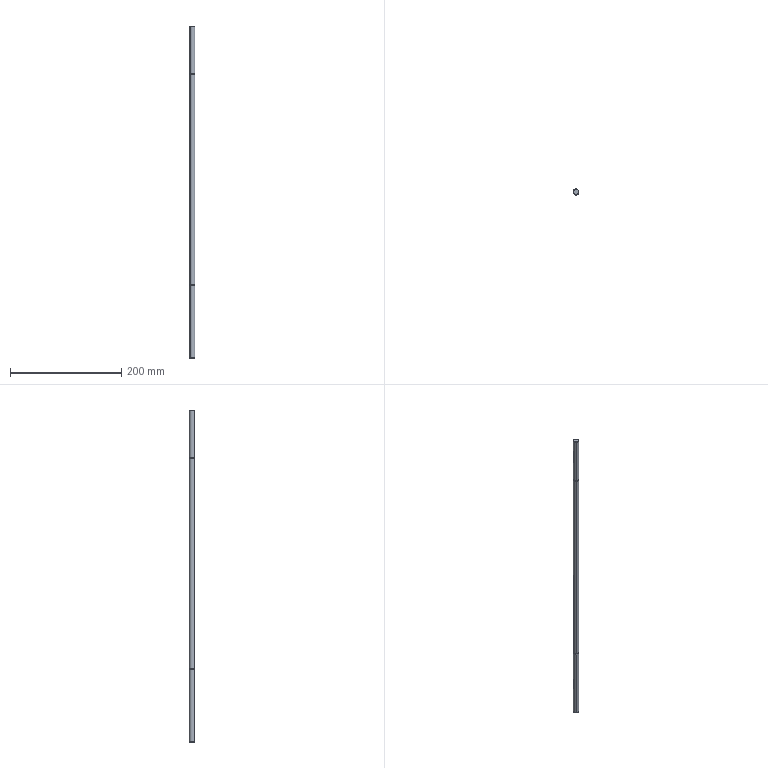Component | SolidWorks | LongGearAxis-1 | 1 solid | 20 faces | box 10 x 10 x 598 mm | volume 46949 mm3 | cylinder 10 | plane 6 | cone 4 | commonest cylinder face diameters 10 x6 9.7 x4
build123d program:
from build123d import *


with BuildPart() as part:
    # Sketch1 → Revolve1 (revolve)
    with BuildSketch(Plane.XY, mode=Mode.PRIVATE) as revolve1_sk:
        Polygon((-299, 4.5), (-299, 0), (299, 0), (299, 4.5), (298.5, 5), (168.6, 5), (168.6, 4.85), (167.5, 4.85), (167.5, 5), (-212.5, 5), (-212.5, 4.85), (-213.6, 4.85), (-213.6, 5), (-298.5, 5), align=None)
    revolve(revolve1_sk.sketch.rotate(Axis((-299, 0, 0), (1, 0, 0)), 270), axis=Axis((-299, 0, 0), (1, 0, 0)))


solid = part.part

# Placed as in the assembly
solid = solid.moved(Location((-180.767, 560.9, -22.5), (0, 90, 0)))
STEP:
#1=CARTESIAN_POINT('',(-7.025,22.234,-12.657));
#2=VERTEX_POINT('',#1);
#3=CARTESIAN_POINT('',(-7.209,21.931,-12.657));
#4=VERTEX_POINT('',#3);
#5=CARTESIAN_POINT('',(-7.117,22.083,-12.657));
#6=DIRECTION('',(0.,-0.,-1.));
#7=DIRECTION('',(0.5208,0.8536,0.));
#8=AXIS2_PLACEMENT_3D('',#5,#6,#7);
#9=CIRCLE('',#8,0.1772);
#10=EDGE_CURVE('',#2,#4,#9,.T.);
#11=ORIENTED_EDGE('',*,*,#10,.F.);
#12=CARTESIAN_POINT('',(-7.014,22.251,-12.638));
#13=VERTEX_POINT('',#12);
#14=CARTESIAN_POINT('',(-7.025,22.234,-12.657));
#15=DIRECTION('',(0.3683,0.6036,0.7071));
#16=VECTOR('',#15,39.37);
#17=LINE('',#14,#16);
#18=EDGE_CURVE('',#2,#13,#17,.T.);
#19=ORIENTED_EDGE('',*,*,#18,.T.);
#20=CARTESIAN_POINT('',(-7.219,21.915,-12.638));
#21=VERTEX_POINT('',#20);
#22=CARTESIAN_POINT('',(-7.117,22.083,-12.638));
#23=DIRECTION('',(0.,-0.,-1.));
#24=DIRECTION('',(0.5208,0.8536,0.));
#25=AXIS2_PLACEMENT_3D('',#22,#23,#24);
#26=CIRCLE('',#25,0.1969);
#27=EDGE_CURVE('',#13,#21,#26,.T.);
#28=ORIENTED_EDGE('',*,*,#27,.T.);
#29=CARTESIAN_POINT('',(-7.209,21.931,-12.657));
#30=DIRECTION('',(-0.3683,-0.6036,0.7071));
#31=VECTOR('',#30,39.37);
#32=LINE('',#29,#31);
#33=EDGE_CURVE('',#4,#21,#32,.T.);
#34=ORIENTED_EDGE('',*,*,#33,.F.);
#35=EDGE_LOOP('',(#11,#19,#28,#34));
#36=FACE_OUTER_BOUND('',#35,.T.);
#37=CARTESIAN_POINT('',(-7.117,22.083,-12.657));
#38=DIRECTION('',(-0.,0.,1.));
#39=DIRECTION('',(-0.5208,-0.8536,0.));
#40=AXIS2_PLACEMENT_3D('',#37,#38,#39);
#41=CONICAL_SURFACE('',#40,0.1772,0.7854);
#42=ADVANCED_FACE('',(#36),#41,.T.);
#43=CARTESIAN_POINT('',(-7.014,22.251,-7.524));
#44=VERTEX_POINT('',#43);
#45=CARTESIAN_POINT('',(-7.219,21.915,-7.524));
#46=VERTEX_POINT('',#45);
#47=CARTESIAN_POINT('',(-7.117,22.083,-7.524));
#48=DIRECTION('',(0.,-0.,-1.));
#49=DIRECTION('',(0.5208,0.8536,0.));
#50=AXIS2_PLACEMENT_3D('',#47,#48,#49);
#51=CIRCLE('',#50,0.1969);
#52=EDGE_CURVE('',#44,#46,#51,.T.);
#53=ORIENTED_EDGE('',*,*,#52,.T.);
#54=CARTESIAN_POINT('',(-7.219,21.915,10.886));
#55=DIRECTION('',(0.,-0.,-1.));
#56=VECTOR('',#55,39.37);
#57=LINE('',#54,#56);
#58=EDGE_CURVE('',#46,#21,#57,.T.);
#59=ORIENTED_EDGE('',*,*,#58,.T.);
#60=ORIENTED_EDGE('',*,*,#27,.F.);
#61=CARTESIAN_POINT('',(-7.014,22.251,10.886));
#62=DIRECTION('',(0.,-0.,-1.));
#63=VECTOR('',#62,39.37);
#64=LINE('',#61,#63);
#65=EDGE_CURVE('',#44,#13,#64,.T.);
#66=ORIENTED_EDGE('',*,*,#65,.F.);
#67=EDGE_LOOP('',(#53,#59,#60,#66));
#68=FACE_OUTER_BOUND('',#67,.T.);
#69=CARTESIAN_POINT('',(-7.117,22.083,10.886));
#70=DIRECTION('',(0.,-0.,-1.));
#71=DIRECTION('',(0.5208,0.8536,0.));
#72=AXIS2_PLACEMENT_3D('',#69,#70,#71);
#73=CYLINDRICAL_SURFACE('',#72,0.1969);
#74=ADVANCED_FACE('',(#68),#73,.T.);
#75=CARTESIAN_POINT('',(-7.017,22.246,-7.48));
#76=VERTEX_POINT('',#75);
#77=CARTESIAN_POINT('',(-7.216,21.92,-7.48));
#78=VERTEX_POINT('',#77);
#79=CARTESIAN_POINT('',(-7.117,22.083,-7.48));
#80=DIRECTION('',(0.,-0.,-1.));
#81=DIRECTION('',(0.5208,0.8536,0.));
#82=AXIS2_PLACEMENT_3D('',#79,#80,#81);
#83=CIRCLE('',#82,0.1909);
#84=EDGE_CURVE('',#76,#78,#83,.T.);
#85=ORIENTED_EDGE('',*,*,#84,.T.);
#86=CARTESIAN_POINT('',(-7.216,21.92,-7.524));
#87=VERTEX_POINT('',#86);
#88=CARTESIAN_POINT('',(-7.216,21.92,10.886));
#89=DIRECTION('',(0.,-0.,-1.));
#90=VECTOR('',#89,39.37);
#91=LINE('',#88,#90);
#92=EDGE_CURVE('',#78,#87,#91,.T.);
#93=ORIENTED_EDGE('',*,*,#92,.T.);
#94=CARTESIAN_POINT('',(-7.017,22.246,-7.524));
#95=VERTEX_POINT('',#94);
#96=CARTESIAN_POINT('',(-7.117,22.083,-7.524));
#97=DIRECTION('',(0.,-0.,-1.));
#98=DIRECTION('',(0.5208,0.8536,0.));
#99=AXIS2_PLACEMENT_3D('',#96,#97,#98);
#100=CIRCLE('',#99,0.1909);
#101=EDGE_CURVE('',#95,#87,#100,.T.);
#102=ORIENTED_EDGE('',*,*,#101,.F.);
#103=CARTESIAN_POINT('',(-7.017,22.246,10.886));
#104=DIRECTION('',(0.,-0.,-1.));
#105=VECTOR('',#104,39.37);
#106=LINE('',#103,#105);
#107=EDGE_CURVE('',#76,#95,#106,.T.);
#108=ORIENTED_EDGE('',*,*,#107,.F.);
#109=EDGE_LOOP('',(#85,#93,#102,#108));
#110=FACE_OUTER_BOUND('',#109,.T.);
#111=CARTESIAN_POINT('',(-7.117,22.083,10.886));
#112=DIRECTION('',(0.,-0.,-1.));
#113=DIRECTION('',(0.5208,0.8536,0.));
#114=AXIS2_PLACEMENT_3D('',#111,#112,#113);
#115=CYLINDRICAL_SURFACE('',#114,0.1909);
#116=ADVANCED_FACE('',(#110),#115,.T.);
#117=CARTESIAN_POINT('',(-7.014,22.251,7.48));
#118=VERTEX_POINT('',#117);
#119=CARTESIAN_POINT('',(-7.219,21.915,7.48));
#120=VERTEX_POINT('',#119);
#121=CARTESIAN_POINT('',(-7.117,22.083,7.48));
#122=DIRECTION('',(0.,-0.,-1.));
#123=DIRECTION('',(0.5208,0.8536,0.));
#124=AXIS2_PLACEMENT_3D('',#121,#122,#123);
#125=CIRCLE('',#124,0.1969);
#126=EDGE_CURVE('',#118,#120,#125,.T.);
#127=ORIENTED_EDGE('',*,*,#126,.T.);
#128=CARTESIAN_POINT('',(-7.219,21.915,-7.48));
#129=VERTEX_POINT('',#128);
#130=CARTESIAN_POINT('',(-7.219,21.915,10.886));
#131=DIRECTION('',(0.,-0.,-1.));
#132=VECTOR('',#131,39.37);
#133=LINE('',#130,#132);
#134=EDGE_CURVE('',#120,#129,#133,.T.);
#135=ORIENTED_EDGE('',*,*,#134,.T.);
#136=CARTESIAN_POINT('',(-7.014,22.251,-7.48));
#137=VERTEX_POINT('',#136);
#138=CARTESIAN_POINT('',(-7.117,22.083,-7.48));
#139=DIRECTION('',(0.,-0.,-1.));
#140=DIRECTION('',(0.5208,0.8536,0.));
#141=AXIS2_PLACEMENT_3D('',#138,#139,#140);
#142=CIRCLE('',#141,0.1969);
#143=EDGE_CURVE('',#137,#129,#142,.T.);
#144=ORIENTED_EDGE('',*,*,#143,.F.);
#145=CARTESIAN_POINT('',(-7.014,22.251,10.886));
#146=DIRECTION('',(0.,-0.,-1.));
#147=VECTOR('',#146,39.37);
#148=LINE('',#145,#147);
#149=EDGE_CURVE('',#118,#137,#148,.T.);
#150=ORIENTED_EDGE('',*,*,#149,.F.);
#151=EDGE_LOOP('',(#127,#135,#144,#150));
#152=FACE_OUTER_BOUND('',#151,.T.);
#153=CARTESIAN_POINT('',(-7.117,22.083,10.886));
#154=DIRECTION('',(0.,-0.,-1.));
#155=DIRECTION('',(0.5208,0.8536,0.));
#156=AXIS2_PLACEMENT_3D('',#153,#154,#155);
#157=CYLINDRICAL_SURFACE('',#156,0.1969);
#158=ADVANCED_FACE('',(#152),#157,.T.);
#159=CARTESIAN_POINT('',(-7.017,22.246,7.524));
#160=VERTEX_POINT('',#159);
#161=CARTESIAN_POINT('',(-7.216,21.92,7.524));
#162=VERTEX_POINT('',#161);
#163=CARTESIAN_POINT('',(-7.117,22.083,7.524));
#164=DIRECTION('',(0.,-0.,-1.));
#165=DIRECTION('',(0.5208,0.8536,0.));
#166=AXIS2_PLACEMENT_3D('',#163,#164,#165);
#167=CIRCLE('',#166,0.1909);
#168=EDGE_CURVE('',#160,#162,#167,.T.);
#169=ORIENTED_EDGE('',*,*,#168,.T.);
#170=CARTESIAN_POINT('',(-7.216,21.92,7.48));
#171=VERTEX_POINT('',#170);
#172=CARTESIAN_POINT('',(-7.216,21.92,10.886));
#173=DIRECTION('',(0.,-0.,-1.));
#174=VECTOR('',#173,39.37);
#175=LINE('',#172,#174);
#176=EDGE_CURVE('',#162,#171,#175,.T.);
#177=ORIENTED_EDGE('',*,*,#176,.T.);
#178=CARTESIAN_POINT('',(-7.017,22.246,7.48));
#179=VERTEX_POINT('',#178);
#180=CARTESIAN_POINT('',(-7.117,22.083,7.48));
#181=DIRECTION('',(0.,-0.,-1.));
#182=DIRECTION('',(0.5208,0.8536,0.));
#183=AXIS2_PLACEMENT_3D('',#180,#181,#182);
#184=CIRCLE('',#183,0.1909);
#185=EDGE_CURVE('',#179,#171,#184,.T.);
#186=ORIENTED_EDGE('',*,*,#185,.F.);
#187=CARTESIAN_POINT('',(-7.017,22.246,10.886));
#188=DIRECTION('',(0.,-0.,-1.));
#189=VECTOR('',#188,39.37);
#190=LINE('',#187,#189);
#191=EDGE_CURVE('',#160,#179,#190,.T.);
#192=ORIENTED_EDGE('',*,*,#191,.F.);
#193=EDGE_LOOP('',(#169,#177,#186,#192));
#194=FACE_OUTER_BOUND('',#193,.T.);
#195=CARTESIAN_POINT('',(-7.117,22.083,10.886));
#196=DIRECTION('',(0.,-0.,-1.));
#197=DIRECTION('',(0.5208,0.8536,0.));
#198=AXIS2_PLACEMENT_3D('',#195,#196,#197);
#199=CYLINDRICAL_SURFACE('',#198,0.1909);
#200=ADVANCED_FACE('',(#194),#199,.T.);
#201=CARTESIAN_POINT('',(-7.014,22.251,10.866));
#202=VERTEX_POINT('',#201);
#203=CARTESIAN_POINT('',(-7.219,21.915,10.866));
#204=VERTEX_POINT('',#203);
#205=CARTESIAN_POINT('',(-7.117,22.083,10.866));
#206=DIRECTION('',(0.,-0.,-1.));
#207=DIRECTION('',(0.5208,0.8536,0.));
#208=AXIS2_PLACEMENT_3D('',#205,#206,#207);
#209=CIRCLE('',#208,0.1969);
#210=EDGE_CURVE('',#202,#204,#209,.T.);
#211=ORIENTED_EDGE('',*,*,#210,.T.);
#212=CARTESIAN_POINT('',(-7.219,21.915,7.524));
#213=VERTEX_POINT('',#212);
#214=CARTESIAN_POINT('',(-7.219,21.915,10.886));
#215=DIRECTION('',(0.,-0.,-1.));
#216=VECTOR('',#215,39.37);
#217=LINE('',#214,#216);
#218=EDGE_CURVE('',#204,#213,#217,.T.);
#219=ORIENTED_EDGE('',*,*,#218,.T.);
#220=CARTESIAN_POINT('',(-7.014,22.251,7.524));
#221=VERTEX_POINT('',#220);
#222=CARTESIAN_POINT('',(-7.117,22.083,7.524));
#223=DIRECTION('',(0.,-0.,-1.));
#224=DIRECTION('',(0.5208,0.8536,0.));
#225=AXIS2_PLACEMENT_3D('',#222,#223,#224);
#226=CIRCLE('',#225,0.1969);
#227=EDGE_CURVE('',#221,#213,#226,.T.);
#228=ORIENTED_EDGE('',*,*,#227,.F.);
#229=CARTESIAN_POINT('',(-7.014,22.251,10.886));
#230=DIRECTION('',(0.,-0.,-1.));
#231=VECTOR('',#230,39.37);
#232=LINE('',#229,#231);
#233=EDGE_CURVE('',#202,#221,#232,.T.);
#234=ORIENTED_EDGE('',*,*,#233,.F.);
#235=EDGE_LOOP('',(#211,#219,#228,#234));
#236=FACE_OUTER_BOUND('',#235,.T.);
#237=CARTESIAN_POINT('',(-7.117,22.083,10.886));
#238=DIRECTION('',(0.,-0.,-1.));
#239=DIRECTION('',(0.5208,0.8536,0.));
#240=AXIS2_PLACEMENT_3D('',#237,#238,#239);
#241=CYLINDRICAL_SURFACE('',#240,0.1969);
#242=ADVANCED_FACE('',(#236),#241,.T.);
#243=CARTESIAN_POINT('',(-7.025,22.234,10.886));
#244=VERTEX_POINT('',#243);
#245=CARTESIAN_POINT('',(-7.209,21.931,10.886));
#246=VERTEX_POINT('',#245);
#247=CARTESIAN_POINT('',(-7.117,22.083,10.886));
#248=DIRECTION('',(0.,-0.,-1.));
#249=DIRECTION('',(0.5208,0.8536,0.));
#250=AXIS2_PLACEMENT_3D('',#247,#248,#249);
#251=CIRCLE('',#250,0.1772);
#252=EDGE_CURVE('',#244,#246,#251,.T.);
#253=ORIENTED_EDGE('',*,*,#252,.T.);
#254=CARTESIAN_POINT('',(-7.219,21.915,10.866));
#255=DIRECTION('',(-0.3683,-0.6036,-0.7071));
#256=VECTOR('',#255,39.37);
#257=LINE('',#254,#256);
#258=EDGE_CURVE('',#246,#204,#257,.T.);
#259=ORIENTED_EDGE('',*,*,#258,.T.);
#260=ORIENTED_EDGE('',*,*,#210,.F.);
#261=CARTESIAN_POINT('',(-7.014,22.251,10.866));
#262=DIRECTION('',(0.3683,0.6036,-0.7071));
#263=VECTOR('',#262,39.37);
#264=LINE('',#261,#263);
#265=EDGE_CURVE('',#244,#202,#264,.T.);
#266=ORIENTED_EDGE('',*,*,#265,.F.);
#267=EDGE_LOOP('',(#253,#259,#260,#266));
#268=FACE_OUTER_BOUND('',#267,.T.);
#269=CARTESIAN_POINT('',(-7.117,22.083,10.866));
#270=DIRECTION('',(0.,-0.,-1.));
#271=DIRECTION('',(0.5208,0.8536,0.));
#272=AXIS2_PLACEMENT_3D('',#269,#270,#271);
#273=CONICAL_SURFACE('',#272,0.1969,0.7854);
#274=ADVANCED_FACE('',(#268),#273,.T.);
#275=ORIENTED_EDGE('',*,*,#258,.F.);
#276=CARTESIAN_POINT('',(-7.117,22.083,10.886));
#277=DIRECTION('',(0.,-0.,-1.));
#278=DIRECTION('',(0.5208,0.8536,0.));
#279=AXIS2_PLACEMENT_3D('',#276,#277,#278);
#280=CIRCLE('',#279,0.1772);
#281=EDGE_CURVE('',#246,#244,#280,.T.);
#282=ORIENTED_EDGE('',*,*,#281,.T.);
#283=ORIENTED_EDGE('',*,*,#265,.T.);
#284=CARTESIAN_POINT('',(-7.117,22.083,10.866));
#285=DIRECTION('',(0.,-0.,-1.));
#286=DIRECTION('',(0.5208,0.8536,0.));
#287=AXIS2_PLACEMENT_3D('',#284,#285,#286);
#288=CIRCLE('',#287,0.1969);
#289=EDGE_CURVE('',#204,#202,#288,.T.);
#290=ORIENTED_EDGE('',*,*,#289,.F.);
#291=EDGE_LOOP('',(#275,#282,#283,#290));
#292=FACE_OUTER_BOUND('',#291,.T.);
#293=CARTESIAN_POINT('',(-7.117,22.083,10.866));
#294=DIRECTION('',(0.,-0.,-1.));
#295=DIRECTION('',(0.5208,0.8536,0.));
#296=AXIS2_PLACEMENT_3D('',#293,#294,#295);
#297=CONICAL_SURFACE('',#296,0.1969,0.7854);
#298=ADVANCED_FACE('',(#292),#297,.T.);
#299=ORIENTED_EDGE('',*,*,#218,.F.);
#300=ORIENTED_EDGE('',*,*,#289,.T.);
#301=ORIENTED_EDGE('',*,*,#233,.T.);
#302=CARTESIAN_POINT('',(-7.117,22.083,7.524));
#303=DIRECTION('',(0.,-0.,-1.));
#304=DIRECTION('',(0.5208,0.8536,0.));
#305=AXIS2_PLACEMENT_3D('',#302,#303,#304);
#306=CIRCLE('',#305,0.1969);
#307=EDGE_CURVE('',#213,#221,#306,.T.);
#308=ORIENTED_EDGE('',*,*,#307,.F.);
#309=EDGE_LOOP('',(#299,#300,#301,#308));
#310=FACE_OUTER_BOUND('',#309,.T.);
#311=CARTESIAN_POINT('',(-7.117,22.083,10.886));
#312=DIRECTION('',(0.,-0.,-1.));
#313=DIRECTION('',(0.5208,0.8536,0.));
#314=AXIS2_PLACEMENT_3D('',#311,#312,#313);
#315=CYLINDRICAL_SURFACE('',#314,0.1969);
#316=ADVANCED_FACE('',(#310),#315,.T.);
#317=ORIENTED_EDGE('',*,*,#227,.T.);
#318=ORIENTED_EDGE('',*,*,#307,.T.);
#319=EDGE_LOOP('',(#317,#318));
#320=FACE_OUTER_BOUND('',#319,.T.);
#321=ORIENTED_EDGE('',*,*,#168,.F.);
#322=CARTESIAN_POINT('',(-7.117,22.083,7.524));
#323=DIRECTION('',(0.,-0.,-1.));
#324=DIRECTION('',(0.5208,0.8536,0.));
#325=AXIS2_PLACEMENT_3D('',#322,#323,#324);
#326=CIRCLE('',#325,0.1909);
#327=EDGE_CURVE('',#162,#160,#326,.T.);
#328=ORIENTED_EDGE('',*,*,#327,.F.);
#329=EDGE_LOOP('',(#321,#328));
#330=FACE_BOUND('',#329,.T.);
#331=CARTESIAN_POINT('',(-6.954,21.983,7.524));
#332=DIRECTION('',(0.,-0.,-1.));
#333=DIRECTION('',(0.5208,0.8536,0.));
#334=AXIS2_PLACEMENT_3D('',#331,#332,#333);
#335=PLANE('',#334);
#336=ADVANCED_FACE('',(#320,#330),#335,.T.);
#337=ORIENTED_EDGE('',*,*,#176,.F.);
#338=ORIENTED_EDGE('',*,*,#327,.T.);
#339=ORIENTED_EDGE('',*,*,#191,.T.);
#340=CARTESIAN_POINT('',(-7.117,22.083,7.48));
#341=DIRECTION('',(0.,-0.,-1.));
#342=DIRECTION('',(0.5208,0.8536,0.));
#343=AXIS2_PLACEMENT_3D('',#340,#341,#342);
#344=CIRCLE('',#343,0.1909);
#345=EDGE_CURVE('',#171,#179,#344,.T.);
#346=ORIENTED_EDGE('',*,*,#345,.F.);
#347=EDGE_LOOP('',(#337,#338,#339,#346));
#348=FACE_OUTER_BOUND('',#347,.T.);
#349=CARTESIAN_POINT('',(-7.117,22.083,10.886));
#350=DIRECTION('',(0.,-0.,-1.));
#351=DIRECTION('',(0.5208,0.8536,0.));
#352=AXIS2_PLACEMENT_3D('',#349,#350,#351);
#353=CYLINDRICAL_SURFACE('',#352,0.1909);
#354=ADVANCED_FACE('',(#348),#353,.T.);
#355=ORIENTED_EDGE('',*,*,#185,.T.);
#356=ORIENTED_EDGE('',*,*,#345,.T.);
#357=EDGE_LOOP('',(#355,#356));
#358=FACE_BOUND('',#357,.T.);
#359=ORIENTED_EDGE('',*,*,#126,.F.);
#360=CARTESIAN_POINT('',(-7.117,22.083,7.48));
#361=DIRECTION('',(0.,-0.,-1.));
#362=DIRECTION('',(0.5208,0.8536,0.));
#363=AXIS2_PLACEMENT_3D('',#360,#361,#362);
#364=CIRCLE('',#363,0.1969);
#365=EDGE_CURVE('',#120,#118,#364,.T.);
#366=ORIENTED_EDGE('',*,*,#365,.F.);
#367=EDGE_LOOP('',(#359,#366));
#368=FACE_OUTER_BOUND('',#367,.T.);
#369=CARTESIAN_POINT('',(-6.949,21.98,7.48));
#370=DIRECTION('',(-0.,0.,1.));
#371=DIRECTION('',(-0.5208,-0.8536,0.));
#372=AXIS2_PLACEMENT_3D('',#369,#370,#371);
#373=PLANE('',#372);
#374=ADVANCED_FACE('',(#358,#368),#373,.T.);
#375=ORIENTED_EDGE('',*,*,#134,.F.);
#376=ORIENTED_EDGE('',*,*,#365,.T.);
#377=ORIENTED_EDGE('',*,*,#149,.T.);
#378=CARTESIAN_POINT('',(-7.117,22.083,-7.48));
#379=DIRECTION('',(0.,-0.,-1.));
#380=DIRECTION('',(0.5208,0.8536,0.));
#381=AXIS2_PLACEMENT_3D('',#378,#379,#380);
#382=CIRCLE('',#381,0.1969);
#383=EDGE_CURVE('',#129,#137,#382,.T.);
#384=ORIENTED_EDGE('',*,*,#383,.F.);
#385=EDGE_LOOP('',(#375,#376,#377,#384));
#386=FACE_OUTER_BOUND('',#385,.T.);
#387=CARTESIAN_POINT('',(-7.117,22.083,10.886));
#388=DIRECTION('',(0.,-0.,-1.));
#389=DIRECTION('',(0.5208,0.8536,0.));
#390=AXIS2_PLACEMENT_3D('',#387,#388,#389);
#391=CYLINDRICAL_SURFACE('',#390,0.1969);
#392=ADVANCED_FACE('',(#386),#391,.T.);
#393=ORIENTED_EDGE('',*,*,#143,.T.);
#394=ORIENTED_EDGE('',*,*,#383,.T.);
#395=EDGE_LOOP('',(#393,#394));
#396=FACE_OUTER_BOUND('',#395,.T.);
#397=ORIENTED_EDGE('',*,*,#84,.F.);
#398=CARTESIAN_POINT('',(-7.117,22.083,-7.48));
#399=DIRECTION('',(0.,-0.,-1.));
#400=DIRECTION('',(0.5208,0.8536,0.));
#401=AXIS2_PLACEMENT_3D('',#398,#399,#400);
#402=CIRCLE('',#401,0.1909);
#403=EDGE_CURVE('',#78,#76,#402,.T.);
#404=ORIENTED_EDGE('',*,*,#403,.F.);
#405=EDGE_LOOP('',(#397,#404));
#406=FACE_BOUND('',#405,.T.);
#407=CARTESIAN_POINT('',(-6.954,21.983,-7.48));
#408=DIRECTION('',(0.,-0.,-1.));
#409=DIRECTION('',(0.5208,0.8536,0.));
#410=AXIS2_PLACEMENT_3D('',#407,#408,#409);
#411=PLANE('',#410);
#412=ADVANCED_FACE('',(#396,#406),#411,.T.);
#413=ORIENTED_EDGE('',*,*,#92,.F.);
#414=ORIENTED_EDGE('',*,*,#403,.T.);
#415=ORIENTED_EDGE('',*,*,#107,.T.);
#416=CARTESIAN_POINT('',(-7.117,22.083,-7.524));
#417=DIRECTION('',(0.,-0.,-1.));
#418=DIRECTION('',(0.5208,0.8536,0.));
#419=AXIS2_PLACEMENT_3D('',#416,#417,#418);
#420=CIRCLE('',#419,0.1909);
#421=EDGE_CURVE('',#87,#95,#420,.T.);
#422=ORIENTED_EDGE('',*,*,#421,.F.);
#423=EDGE_LOOP('',(#413,#414,#415,#422));
#424=FACE_OUTER_BOUND('',#423,.T.);
#425=CARTESIAN_POINT('',(-7.117,22.083,10.886));
#426=DIRECTION('',(0.,-0.,-1.));
#427=DIRECTION('',(0.5208,0.8536,0.));
#428=AXIS2_PLACEMENT_3D('',#425,#426,#427);
#429=CYLINDRICAL_SURFACE('',#428,0.1909);
#430=ADVANCED_FACE('',(#424),#429,.T.);
#431=ORIENTED_EDGE('',*,*,#101,.T.);
#432=ORIENTED_EDGE('',*,*,#421,.T.);
#433=EDGE_LOOP('',(#431,#432));
#434=FACE_BOUND('',#433,.T.);
#435=ORIENTED_EDGE('',*,*,#52,.F.);
#436=CARTESIAN_POINT('',(-7.117,22.083,-7.524));
#437=DIRECTION('',(0.,-0.,-1.));
#438=DIRECTION('',(0.5208,0.8536,0.));
#439=AXIS2_PLACEMENT_3D('',#436,#437,#438);
#440=CIRCLE('',#439,0.1969);
#441=EDGE_CURVE('',#46,#44,#440,.T.);
#442=ORIENTED_EDGE('',*,*,#441,.F.);
#443=EDGE_LOOP('',(#435,#442));
#444=FACE_OUTER_BOUND('',#443,.T.);
#445=CARTESIAN_POINT('',(-6.949,21.98,-7.524));
#446=DIRECTION('',(-0.,0.,1.));
#447=DIRECTION('',(-0.5208,-0.8536,0.));
#448=AXIS2_PLACEMENT_3D('',#445,#446,#447);
#449=PLANE('',#448);
#450=ADVANCED_FACE('',(#434,#444),#449,.T.);
#451=ORIENTED_EDGE('',*,*,#58,.F.);
#452=ORIENTED_EDGE('',*,*,#441,.T.);
#453=ORIENTED_EDGE('',*,*,#65,.T.);
#454=CARTESIAN_POINT('',(-7.117,22.083,-12.638));
#455=DIRECTION('',(0.,-0.,-1.));
#456=DIRECTION('',(0.5208,0.8536,0.));
#457=AXIS2_PLACEMENT_3D('',#454,#455,#456);
#458=CIRCLE('',#457,0.1969);
#459=EDGE_CURVE('',#21,#13,#458,.T.);
#460=ORIENTED_EDGE('',*,*,#459,.F.);
#461=EDGE_LOOP('',(#451,#452,#453,#460));
#462=FACE_OUTER_BOUND('',#461,.T.);
#463=CARTESIAN_POINT('',(-7.117,22.083,10.886));
#464=DIRECTION('',(0.,-0.,-1.));
#465=DIRECTION('',(0.5208,0.8536,0.));
#466=AXIS2_PLACEMENT_3D('',#463,#464,#465);
#467=CYLINDRICAL_SURFACE('',#466,0.1969);
#468=ADVANCED_FACE('',(#462),#467,.T.);
#469=ORIENTED_EDGE('',*,*,#18,.F.);
#470=CARTESIAN_POINT('',(-7.117,22.083,-12.657));
#471=DIRECTION('',(0.,-0.,-1.));
#472=DIRECTION('',(0.5208,0.8536,0.));
#473=AXIS2_PLACEMENT_3D('',#470,#471,#472);
#474=CIRCLE('',#473,0.1772);
#475=EDGE_CURVE('',#4,#2,#474,.T.);
#476=ORIENTED_EDGE('',*,*,#475,.F.);
#477=ORIENTED_EDGE('',*,*,#33,.T.);
#478=ORIENTED_EDGE('',*,*,#459,.T.);
#479=EDGE_LOOP('',(#469,#476,#477,#478));
#480=FACE_OUTER_BOUND('',#479,.T.);
#481=CARTESIAN_POINT('',(-7.117,22.083,-12.657));
#482=DIRECTION('',(-0.,0.,1.));
#483=DIRECTION('',(-0.5208,-0.8536,0.));
#484=AXIS2_PLACEMENT_3D('',#481,#482,#483);
#485=CONICAL_SURFACE('',#484,0.1772,0.7854);
#486=ADVANCED_FACE('',(#480),#485,.T.);
#487=ORIENTED_EDGE('',*,*,#475,.T.);
#488=ORIENTED_EDGE('',*,*,#10,.T.);
#489=EDGE_LOOP('',(#487,#488));
#490=FACE_OUTER_BOUND('',#489,.T.);
#491=CARTESIAN_POINT('',(-7.117,22.083,-12.657));
#492=DIRECTION('',(0.,-0.,-1.));
#493=DIRECTION('',(0.5208,0.8536,0.));
#494=AXIS2_PLACEMENT_3D('',#491,#492,#493);
#495=PLANE('',#494);
#496=ADVANCED_FACE('',(#490),#495,.T.);
#497=ORIENTED_EDGE('',*,*,#252,.F.);
#498=ORIENTED_EDGE('',*,*,#281,.F.);
#499=EDGE_LOOP('',(#497,#498));
#500=FACE_OUTER_BOUND('',#499,.T.);
#501=CARTESIAN_POINT('',(-6.966,21.99,10.886));
#502=DIRECTION('',(-0.,0.,1.));
#503=DIRECTION('',(-0.5208,-0.8536,0.));
#504=AXIS2_PLACEMENT_3D('',#501,#502,#503);
#505=PLANE('',#504);
#506=ADVANCED_FACE('',(#500),#505,.T.);
#507=CLOSED_SHELL('',(#42,#74,#116,#158,#200,#242,#274,#298,#316,#336,#354,#374,#392,#412,#430,#450,#468,#486,#496,#506));
#508=MANIFOLD_SOLID_BREP('',#507);
#509=CARTESIAN_POINT('',(0.,0.,0.));
#510=DIRECTION('',(0.,0.,1.));
#511=DIRECTION('',(1.,0.,0.));
#512=AXIS2_PLACEMENT_3D('',#509,#510,#511);
#513=(LENGTH_UNIT()NAMED_UNIT(*)SI_UNIT($,.METRE.));
#514=LENGTH_MEASURE_WITH_UNIT(LENGTH_MEASURE(0.0254),#513);
#515=DIMENSIONAL_EXPONENTS(1.,0.,0.,0.,0.,0.,0.);
#516=(CONVERSION_BASED_UNIT('',#514)LENGTH_UNIT()NAMED_UNIT(#515));
#517=UNCERTAINTY_MEASURE_WITH_UNIT(LENGTH_MEASURE(0.00001),#516,'','');
#518=(NAMED_UNIT(*)PLANE_ANGLE_UNIT()SI_UNIT($,.RADIAN.));
#519=(NAMED_UNIT(*)SI_UNIT($,.STERADIAN.)SOLID_ANGLE_UNIT());
#520=(GEOMETRIC_REPRESENTATION_CONTEXT(3)GLOBAL_UNCERTAINTY_ASSIGNED_CONTEXT((#517))GLOBAL_UNIT_ASSIGNED_CONTEXT((#516,#518,#519))REPRESENTATION_CONTEXT('',''));
#521=ADVANCED_BREP_SHAPE_REPRESENTATION('',(#508,#512),#520);
#522=COLOUR_RGB('',0.7922,0.8196,0.9333);
#523=FILL_AREA_STYLE_COLOUR('',#522);
#524=FILL_AREA_STYLE('',(#523));
#525=SURFACE_STYLE_FILL_AREA(#524);
#526=SURFACE_SIDE_STYLE('',(#525));
#527=SURFACE_STYLE_USAGE(.BOTH.,#526);
#528=PRESENTATION_STYLE_ASSIGNMENT((#527));
#529=STYLED_ITEM('',(#528),#508);
#530=PRESENTATION_LAYER_ASSIGNMENT('','',(#529));
#531=(LENGTH_UNIT()NAMED_UNIT(*)SI_UNIT($,.METRE.));
#532=LENGTH_MEASURE_WITH_UNIT(LENGTH_MEASURE(0.0254),#531);
#533=DIMENSIONAL_EXPONENTS(1.,0.,0.,0.,0.,0.,0.);
#534=(CONVERSION_BASED_UNIT('',#532)LENGTH_UNIT()NAMED_UNIT(#533));
#535=UNCERTAINTY_MEASURE_WITH_UNIT(LENGTH_MEASURE(0.00001),#534,'','');
#536=(NAMED_UNIT(*)PLANE_ANGLE_UNIT()SI_UNIT($,.RADIAN.));
#537=(NAMED_UNIT(*)SI_UNIT($,.STERADIAN.)SOLID_ANGLE_UNIT());
#538=(GEOMETRIC_REPRESENTATION_CONTEXT(3)GLOBAL_UNCERTAINTY_ASSIGNED_CONTEXT((#535))GLOBAL_UNIT_ASSIGNED_CONTEXT((#534,#536,#537))REPRESENTATION_CONTEXT('',''));
#539=MECHANICAL_DESIGN_GEOMETRIC_PRESENTATION_REPRESENTATION('',(#529),#538);